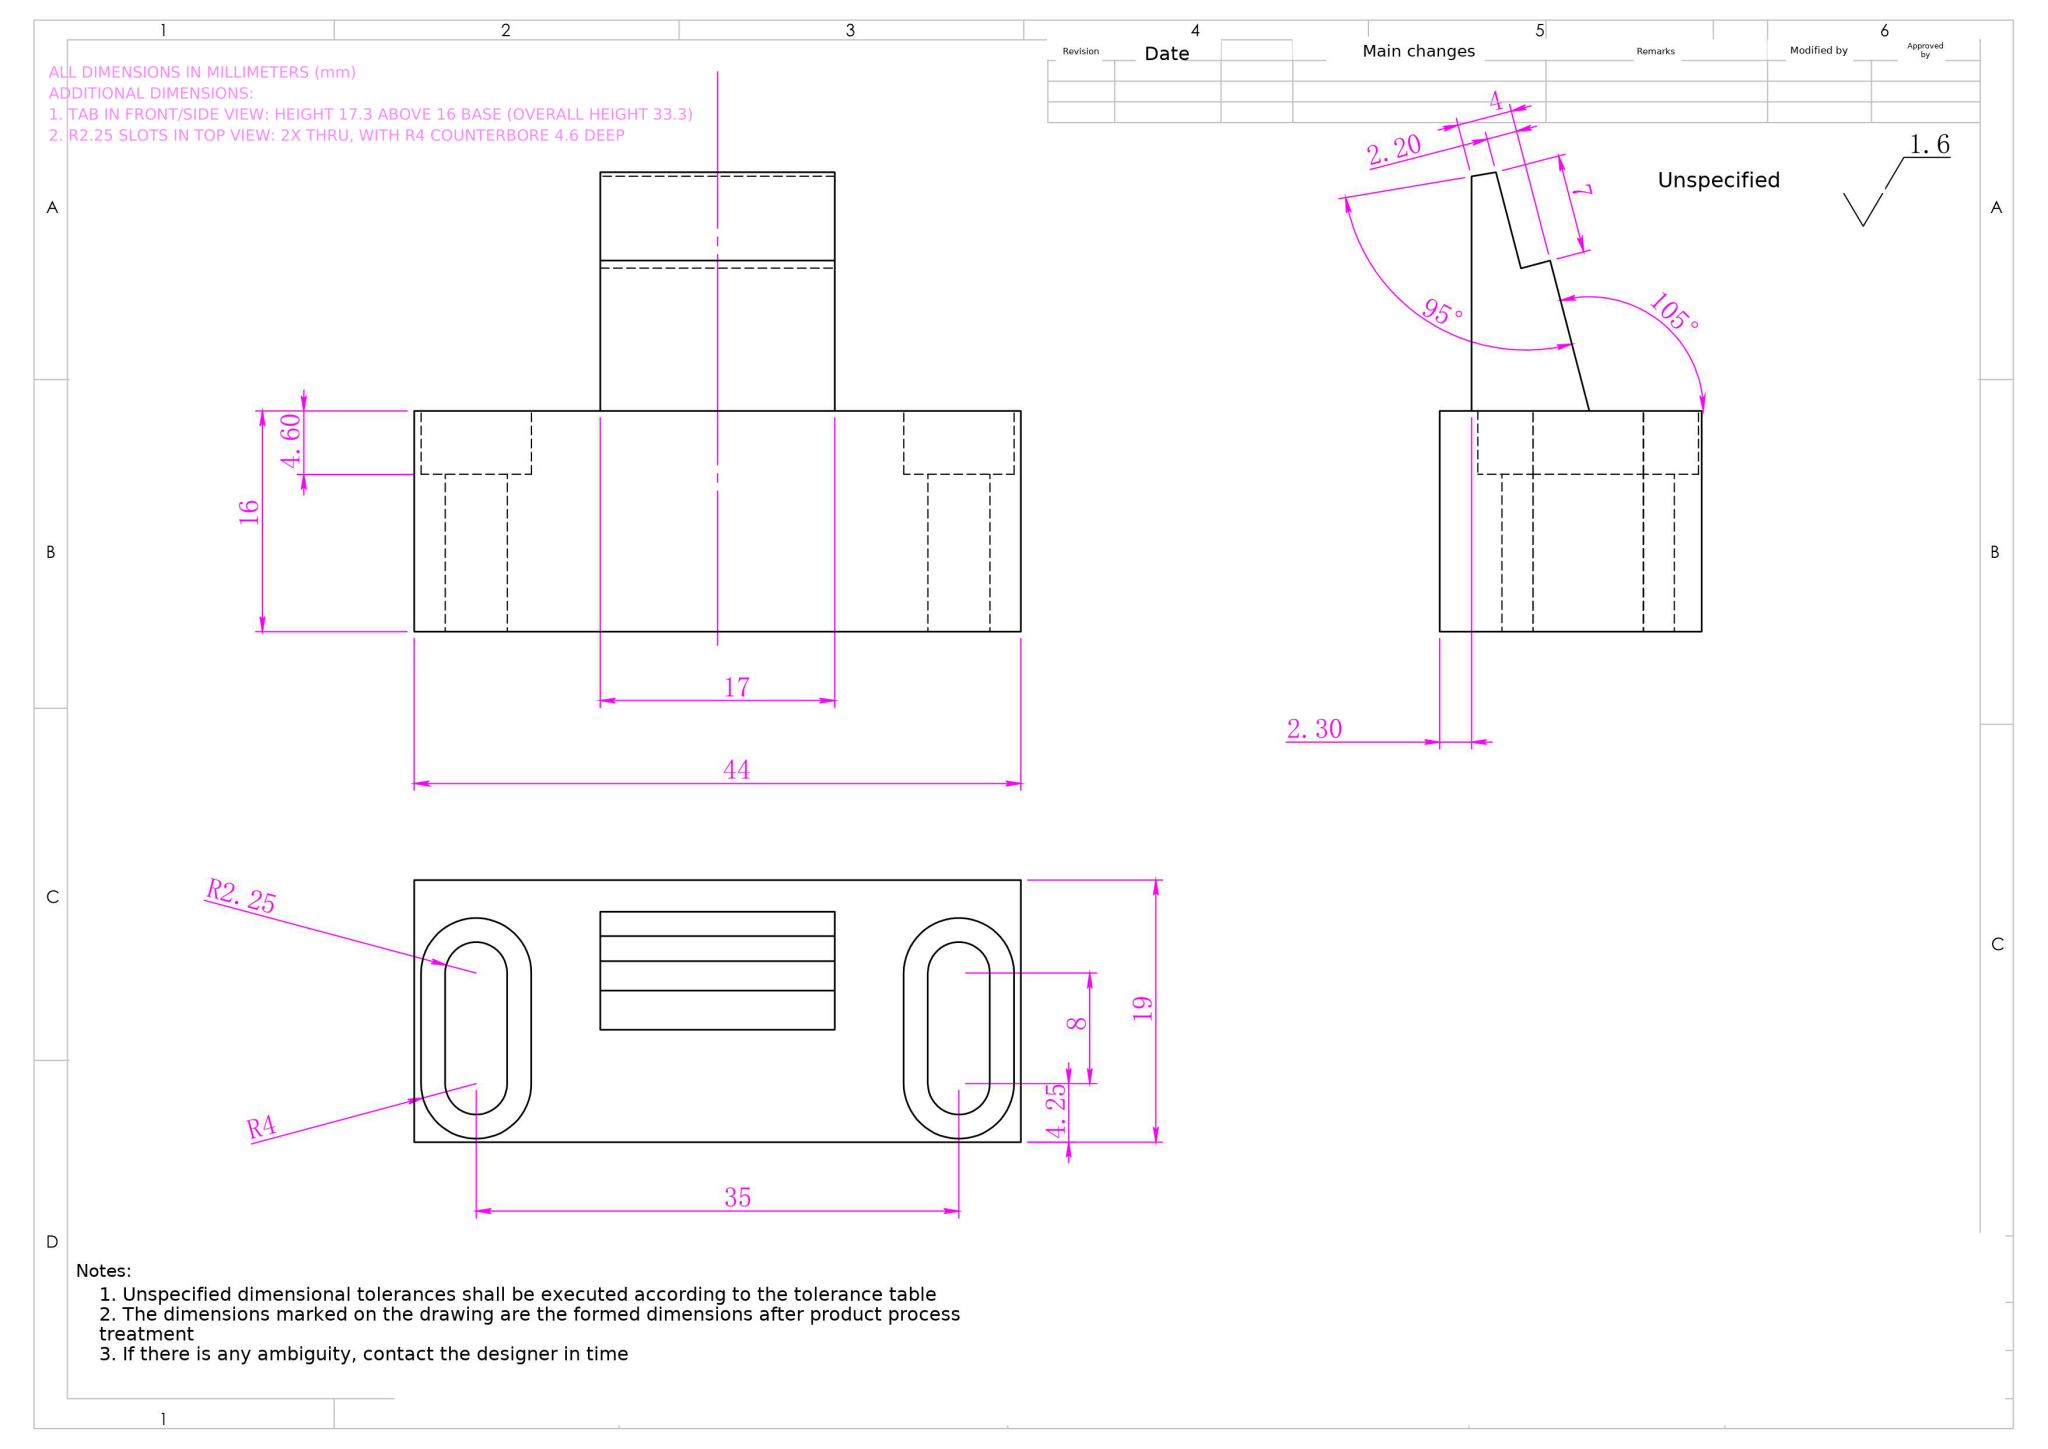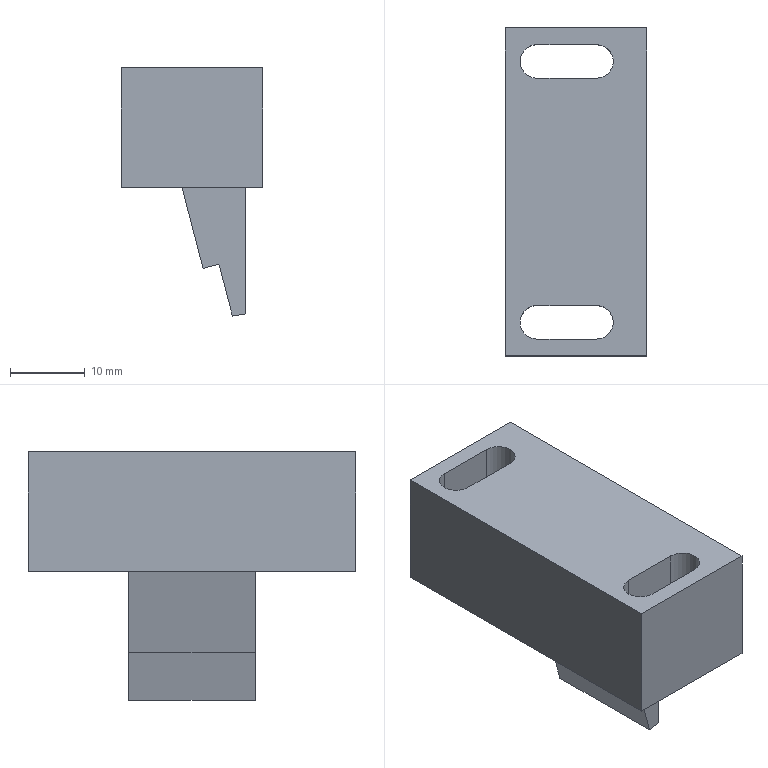Part | NX | mm | 1 solid | 35 faces | box 19 x 44 x 33.3 mm | volume 12729 mm3 | plane 23 | cylinder 12 | commonest cylinder face diameters 8 x6 4.5 x6